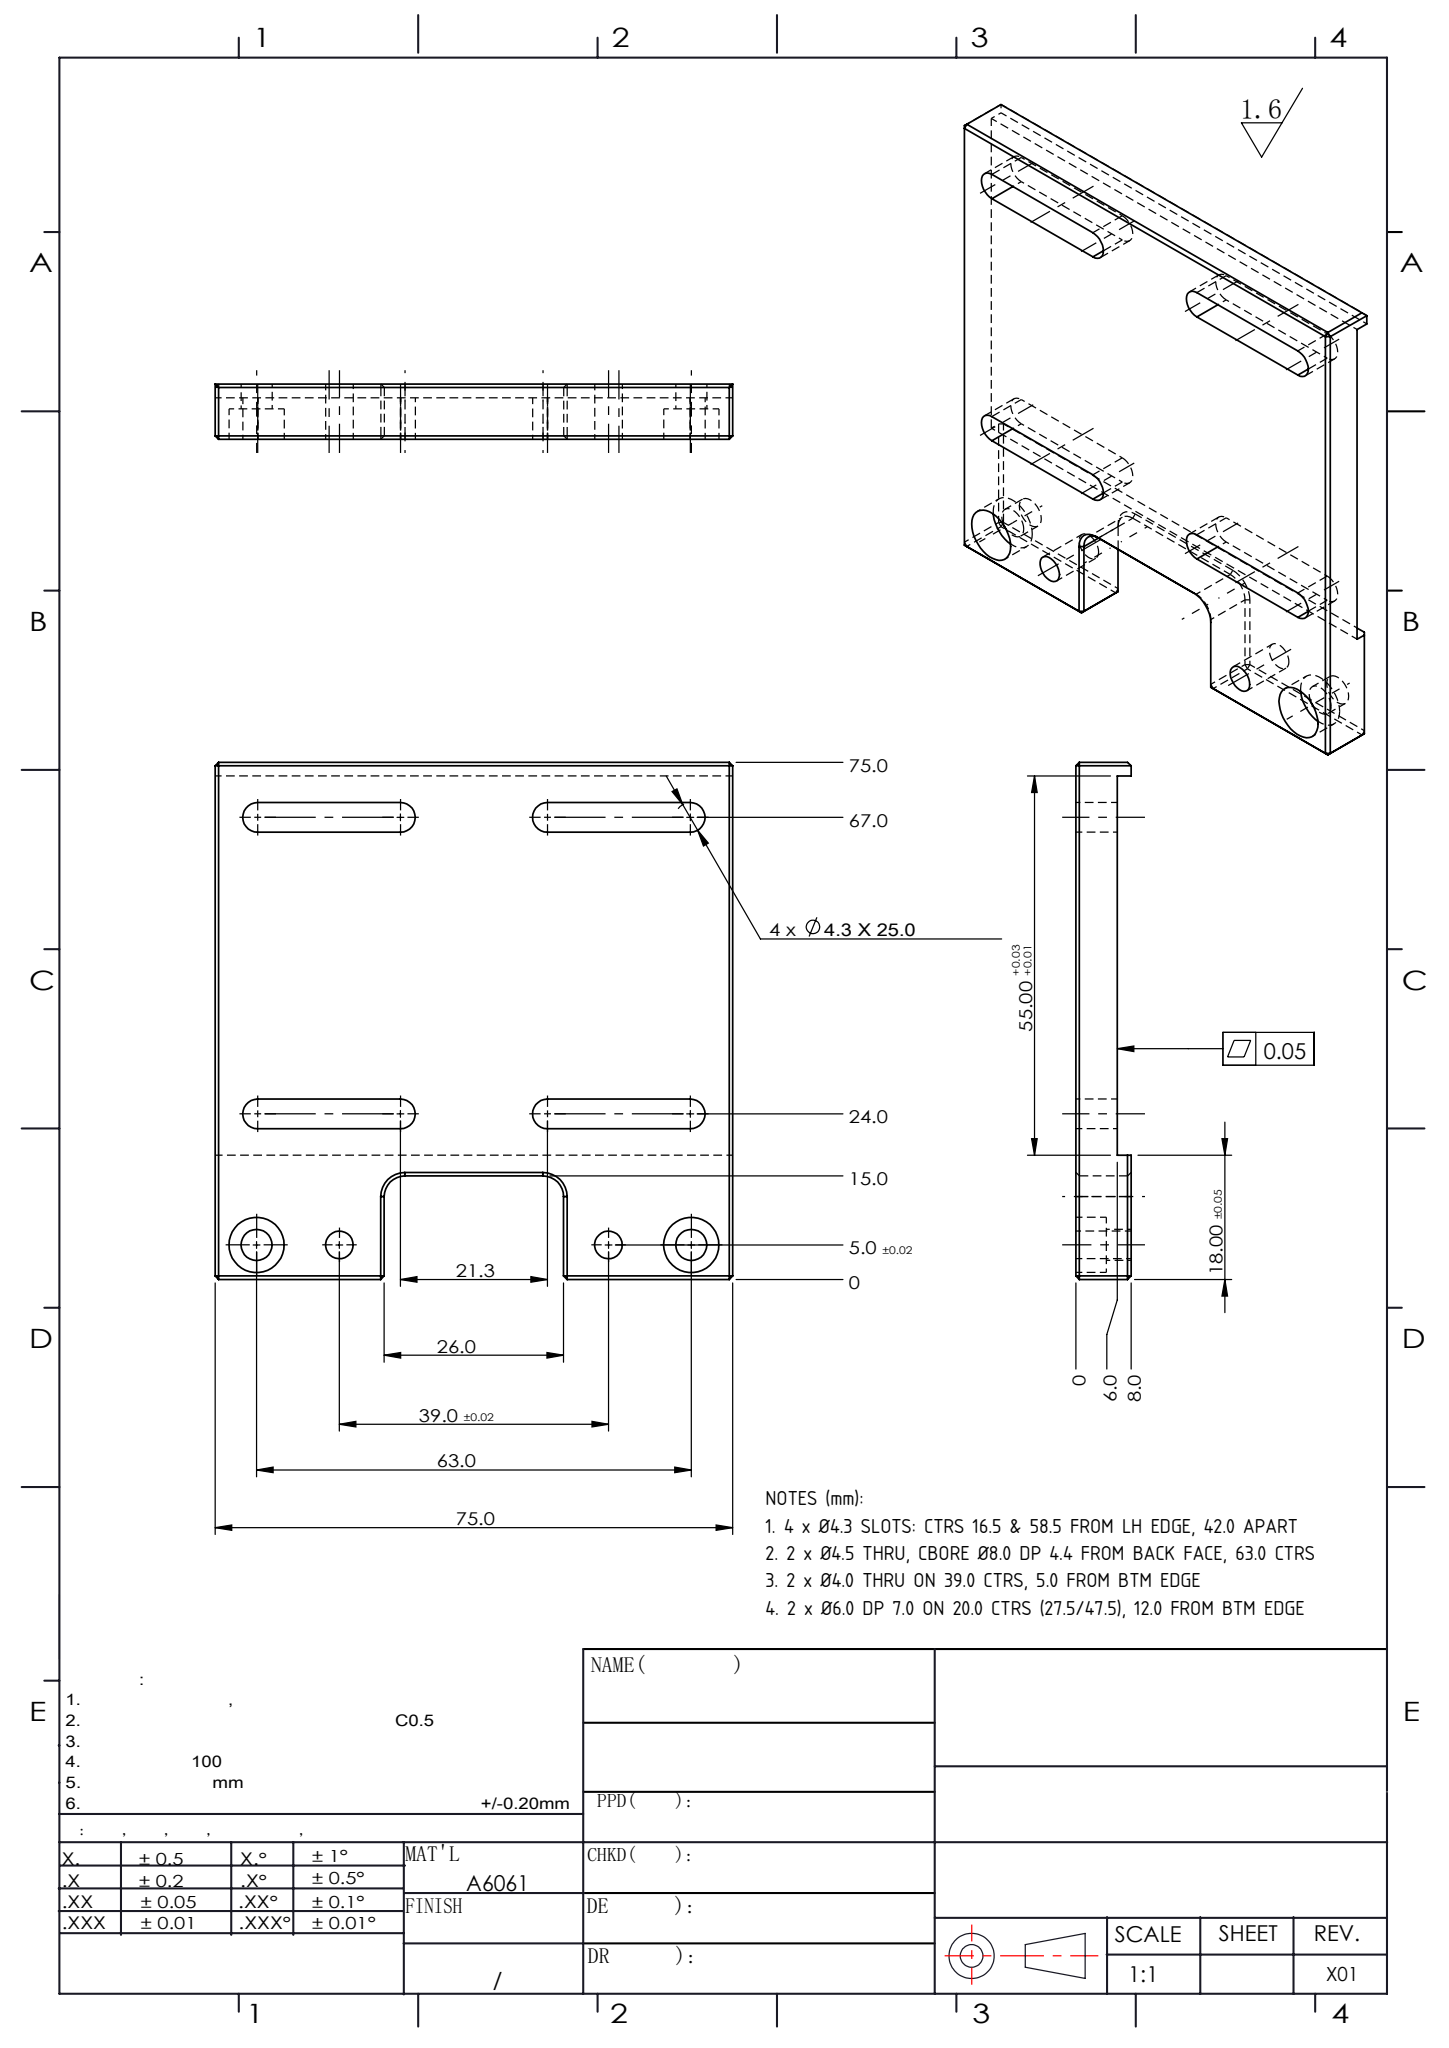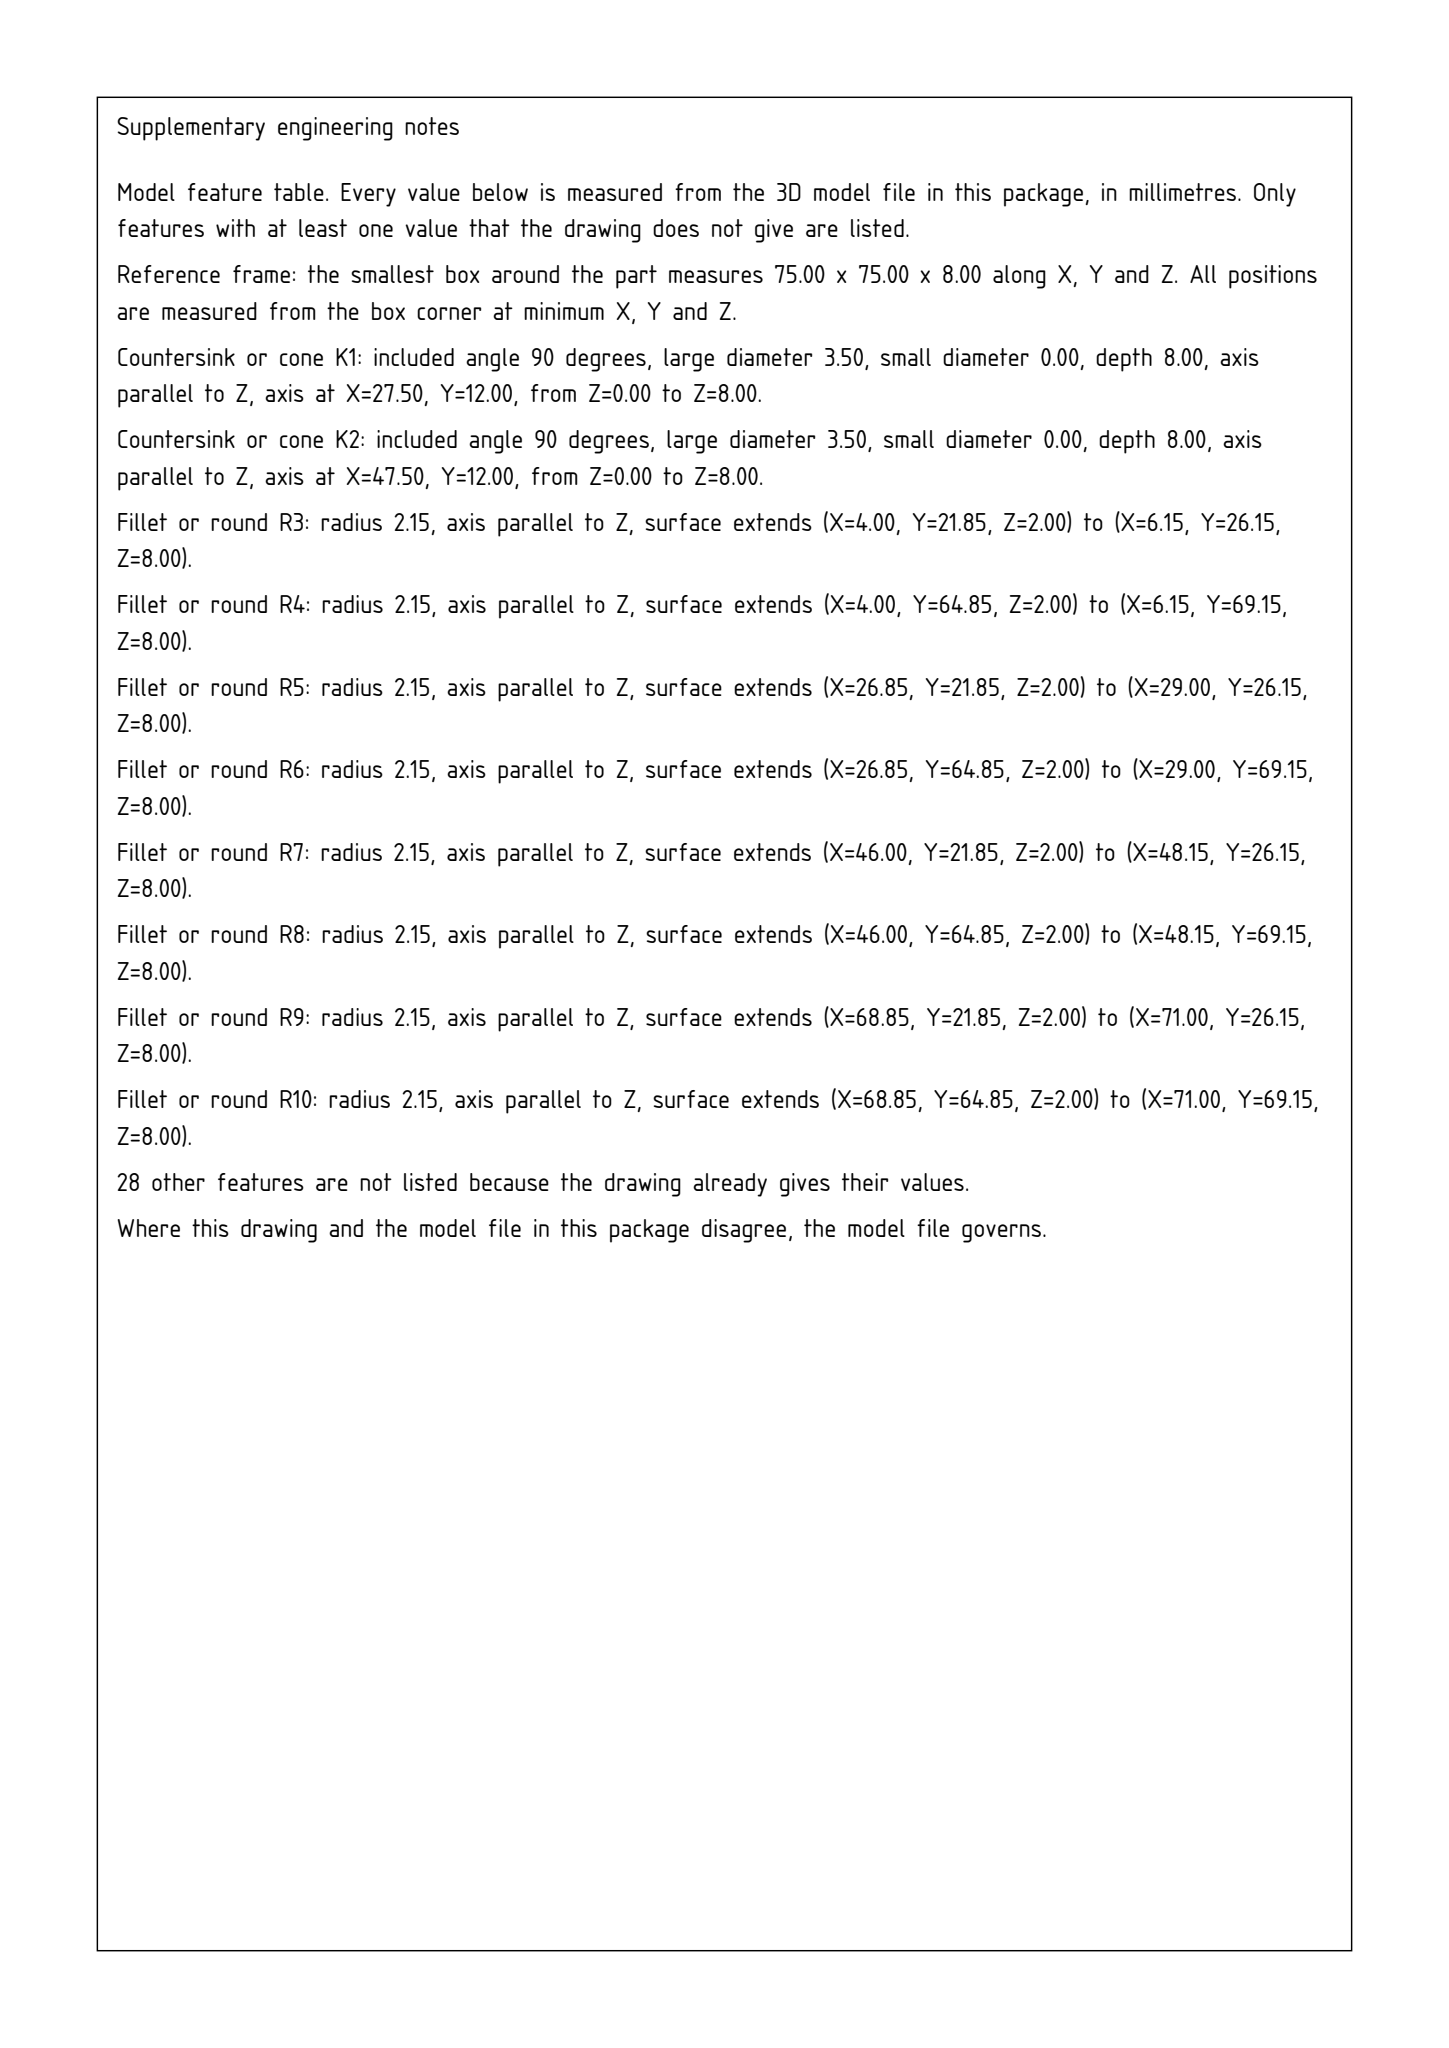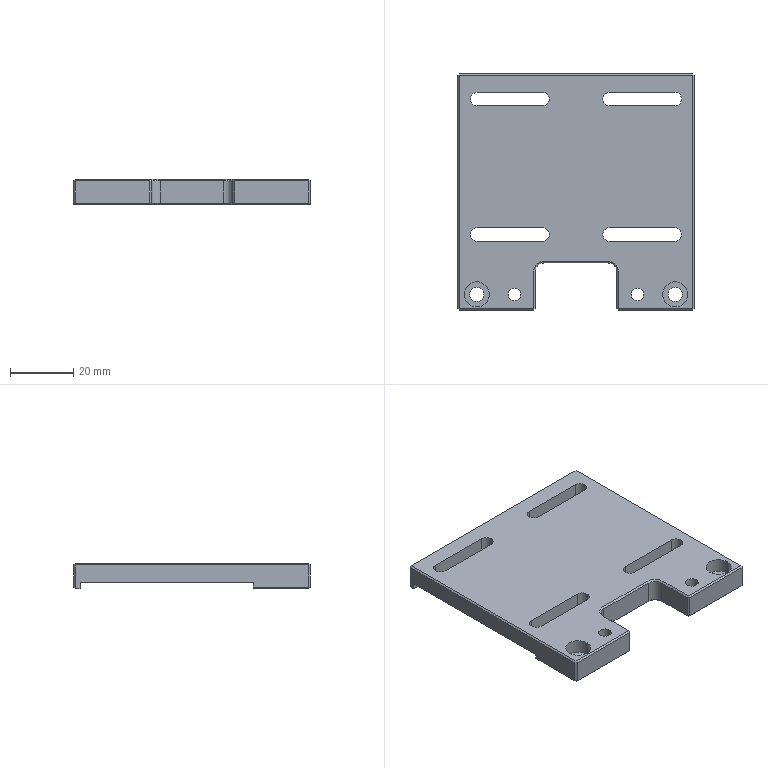Part | SolidWorks | mm | 1 solid | 86 faces | box 75 x 75 x 8 mm | volume 30345 mm3 | plane 56 | cylinder 26 | cone 4 | commonest cylinder face diameters 4.3 x12 4 x4 8 x4 4.5 x4 6 x2
Drawing notes:
4 x Ø4.3 SLOTS: CTRS 16.5 & 58.5 FROM LH EDGE, 42.0 APART | from the solid: Ø4.3 end cyls at X=6.15/26.85 and 48.15/68.85 (ctrs 16.5 & 58.5, 25.0 slot lg)
2 x Ø4.5 THRU, CBORE Ø8.0 DP 4.4 FROM BACK FACE, 63.0 CTRS | from the solid: Ø4.5 L3.6 at X=6.0/69.0 Y=5.0; Ø8.0 L4.4 same axes (8.0 plate thk)
2 x Ø4.0 THRU ON 39.0 CTRS, 5.0 FROM BTM EDGE | from the solid: Ø4.0 z-cyls, L8.0 (thru), at X=18.0 & 57.0, Y=5.0
2 x Ø6.0 DP 7.0 ON 20.0 CTRS (27.5/47.5), 12.0 FROM BTM EDGE | from the solid: Ø6.0 z-cyls L7.0 at X=27.5 & 47.5, Y=12.0